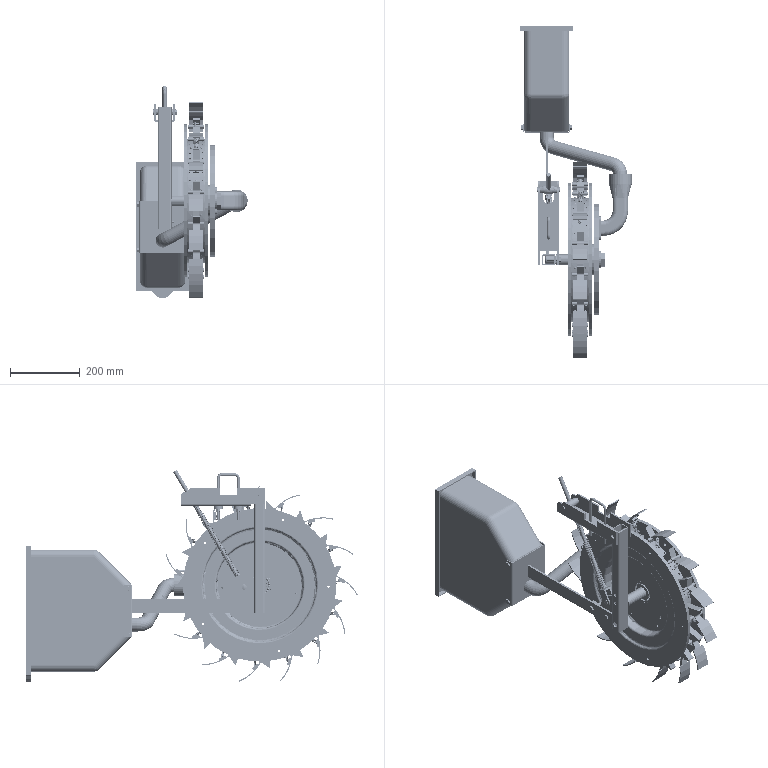Assembly | SolidWorks | mm | 152 component files | 153 solids | 5112 faces | box 318.78 x 951.87 x 608.54 mm | volume 5125266 mm3 | plane 2818 | cylinder 1742 | sphere 196 | torus 194 | cone 118 | spline 44 | commonest cylinder face diameters 3 x287 6 x230 10 x204 0.2 x184 5 x122 5.6 x92 234 x60 9 x58
Bill of materials:
10x25DowelPin | 1 |  | Solid cylindrical pin with a larger-diameter disc head at each end; the outer faces of both heads are slightly domed.
8x50U-Bolt | 1 |  | Round wire or rod bent into a U shape: two straight parallel legs joined by a straight crossbar with rounded bends; one leg is visibly shorter.
hex slotted nuts style 1-grades c gb | 2 |  | Hexagonal nut-like body with a central through bore and radial round-ended slots cut into one end face (castellated form).
hexagon head bolts-full thread gb | 7 |  | Hex-head bolt-like part with a plain cylindrical shank and a chamfered tip.
PullRod | 1 |  | Long slender round rod ending in a forked clevis-style block with two parallel tines, each with a cross hole.
SeedBox | 1 |  | Hollow box-shaped housing or cover with rounded edges, one chamfered (angled) top corner, an open flanged end, and a small cylindrical boss/spigot on one side.
SeedBoxBracket | 1 |  | Sheet-metal bracket: a channel-shaped mounting plate with bent side flanges, plus a long flat arm projecting perpendicular from its face.
SeedBoxCover | 1 |  | Thin flat rectangular plate with a semicircular tab or lobe protruding from the middle of one short edge.
SeederBracket | 1 |  | Rectangular hollow tube post with holes along its length and a flat gusset-like plate with a lobed outline attached near the bottom.
SeederFixingFrame | 1 |  | U-shaped sheet-metal channel bracket with two parallel side plates of stepped height and a connecting web.
16008 Bearing | 2 |  | Ring-shaped assembly resembling a radial ball bearing: concentric inner and outer rings with a ring of spherical elements between them.
cross recessed pan head screws gb | 46 |  | Pan-head screw-like part with a cross-shaped recess in a domed cylindrical head and a plain cylindrical shank.
Duckbill | 15 |  | Thin rectangular base plate curved in one direction, carrying an inclined hollow rectangular column with an open top, a cylindrical knuckle with a bore on the column, and a small tab with an upright cylindrical pin.
DuckbillSpring | 15 |  | Helical coil of round-section wire with a constant coil diameter, roughly 12-13 evenly pitched turns and plain cut ends.
PressingPlate | 15 |  | Thin formed sheet piece: a long curved strip joined at a V-shaped bend to a short straight flange. Hollow cylindrical knuckle(s) sit at the bend, and a rectangular raised pad is on the strip near the bend.
SeedingAxis | 1 |  | Stepped cylindrical pin with a hexagonal head, a thin round collar under the head, a long main shank and a shorter reduced-diameter end section.
SeedingFixingPlate | 1 |  | Large thin circular disc with a central through-bore and stepped concentric cylindrical hub bosses on one face. There is a shallow circular ridge or groove near the rim and two rings of small holes.
SeedingFixingPlateA | 1 |  | Flat annular ring with a stepped cross-section: a thin full-diameter flange plus a thicker layer of smaller outer diameter. It has a large central opening and five small holes on a circle.
SeedingPlate | 1 |  | Thin circular disc with a central round hole and a short cylindrical boss at the center on one face. It has an off-center rounded-square cutout ringed by four small holes, and six small holes near the rim.
SeedingSlot | 15 |  | Complex bracket built around a flat, roughly hexagonal plate with two end lugs that carry cylindrical bosses with through-holes. One side has a rectangular hollow frame or box; the other has an angled hollow channel with a partly cylindrical inner surface and a tapered internal transition.
SeedInlet | 1 |  | Flanged duct: a rectangular flange with rounded corners and four holes leads into a rounded-rectangle duct that bends about 90 degrees, then changes to a larger round section at the far end.
SeedSpoonPlate | 15 |  | Central disc hub with a through-bore. Arms run outward in four directions and end in cylindrical shells of different sizes; some are open semi-cylinders or tubes.
SeedTube | 1 |  | Hollow round tube with two bends forming an offset jog between three straight sections, open at both ends.
ShaftStop | 1 |  | Solid barrel-shaped body bulging in the middle, with a smaller cylindrical spigot at each end and a radial cross-hole through the middle of the body.
single coil spring lock washers heavy gb | 4 |  | Flat annular ring with rectangular cross-section, split by a single narrow radial cut whose faces are angled; resembles a split (helical spring) lock washer.
Spring2 | 1 |  | Long, slender helical coil spring of round wire with constant diameter and many evenly spaced coils; resembles an open-coil compression spring.
Mates:
1. concentric | SeederFixingFrame-1 face at (-210, -105, 2.5) dir (1, 0, 0) r 6 | SeederBracket-1 face at (-20, -105, 2.5) dir (1, 0, 0) r 6
2. coincident | SeederBracket-1 plane at (0, -105, -157.5) dir (1, 0, 0) | assembly plane at (0, 0, 0) dir (1, 0, 0)
3. concentric | SeederFixingFrame-1 face at (-210, -105, 2.5) dir (1, 0, 0) r 6 | hexagon head bolts-full thread gb-1 face at (-5, -105, 2.5) dir (1, 0, 0) r 4
4. coincident | SeederFixingFrame-1 face at (30, 120, 25) dir (1, 0, 0) | hexagon head bolts-full thread gb-1 face at (30, -109.574, -3.45) dir (-1, 0, 0)
5. concentric | SeederFixingFrame-1 face at (-30, 95, 2.5) dir (1, 0, 0) r 7.5 | ShaftStop-1 face at (33, 95, 2.5) dir (-1, 0, 0) r 7.5
6. coincident | ShaftStop-1 plane at (0, 95, 2.5) dir (1, 0, 0) | assembly plane at (0, 0, 0) dir (1, 0, 0)
7. concentric | SeederBracket-1 face at (-2.5, -60.308, -258.214) dir (1, 0, 0) r 5 | PullRod-1 face at (-12.5, -60.308, -258.214) dir (1, 0, 0) r 5
8. concentric | ShaftStop-1 face at (0, 103.444, 16.675) dir (0, -0.5118, -0.8591) r 6 | PullRod-1 face at (0, 138.006, 74.694) dir (0, -0.5118, -0.8591) r 6
9. concentric | PullRod-1 face at (0, 138.006, 74.694) dir (0, -0.5118, -0.8591) r 6 | Spring2-1 sketch segment at (0, -41.116, -225.997) dir (0, 0.5118, 0.8591) r 7.5
10. coincident | PullRod-1 face at (12.5, -30.377, -232.395) dir (0, 0.5118, 0.8591) | Spring2-1 face at (0, -41.116, -225.997) dir (0, -0.5118, -0.8591)
11. concentric | PullRod-1 face at (-12.5, -60.308, -258.214) dir (1, 0, 0) r 5 | 10x25DowelPin-1 face at (14.5, -60.308, -258.214) dir (-1, 0, 0) r 7.5
12. coincident | PullRod-1 face at (12.5, 48.445, -75.652) dir (1, 0, 0) | 10x25DowelPin-1 face at (12.5, -60.308, -258.214) dir (-1, 0, 0)
13. coincident | SeederBracket-1 face at (-2.5, 21.34, -327.5) dir (-1, 0, 0) | SeedBoxBracket-1 face at (-2.5, -90, -292.5) dir (1, 0, 0)
14. concentric | SeederBracket-1 face at (-2.5, -60, -312.5) dir (1, 0, 0) r 5 | SeedBoxBracket-1 face at (-402.5, -60, -312.5) dir (1, 0, 0) r 5
15. concentric | SeederBracket-1 face at (-2.5, 0, -312.5) dir (1, 0, 0) r 5 | SeedBoxBracket-1 face at (-402.5, 0, -312.5) dir (1, 0, 0) r 5
16. concentric | SeedBoxBracket-1 face at (-402.5, -60, -312.5) dir (1, 0, 0) r 5 | hexagon head bolts-full thread gb-2 face at (26.5, -60, -312.5) dir (-1, 0, 0) r 4
17. coincident | SeedBoxBracket-1 face at (-8.5, -90, -292.5) dir (-1, 0, 0) | hexagon head bolts-full thread gb-2 face at (-8.5, -63.753, -319) dir (1, 0, 0)
18. concentric | SeedBoxBracket-1 face at (-402.5, 0, -312.5) dir (1, 0, 0) r 5 | hexagon head bolts-full thread gb-3 face at (26.5, 0, -312.5) dir (-1, 0, 0) r 4
19. coincident | SeedBoxBracket-1 face at (-8.5, -90, -292.5) dir (-1, 0, 0) | hexagon head bolts-full thread gb-3 face at (-8.5, -3.753, -319) dir (1, 0, 0)
20. coincident | SeedBoxBracket-1 face at (57.5, 262.5, -402.5) dir (0, 1, 0) | SeedBox-1 face at (59.5, 262.5, -401.036) dir (0, -1, 0)
21. coincident | SeedBoxBracket-1 face at (59.5, 285, -402.5) dir (-1, 0, 0) | SeedBox-1 face at (59.5, 262.5, -326.036) dir (1, 0, 0)
22. coincident | SeedBoxBracket-1 face at (-68.5, 264.5, -402.5) dir (0, 0, -1) | SeedBox-1 edge at (39.5, 263.964, -402.5) dir (-1, 0, 0)
23. coincident | SeedBoxBracket-1 face at (62, 285, -402.5) dir (1, 0, 0) | hexagon head bolts-full thread gb-4 face at (62, 279.324, -256.55) dir (-1, 0, 0)
24. concentric | SeedBoxBracket-1 face at (-73, 274.75, -262.5) dir (1, 0, 0) r 4.5 | hexagon head bolts-full thread gb-4 face at (27, 274.75, -262.5) dir (1, 0, 0) r 4
25. concentric | SeedBoxBracket-1 face at (-73, 274.75, -392.5) dir (1, 0, 0) r 4.5 | hexagon head bolts-full thread gb-5 face at (27, 274.75, -392.5) dir (1, 0, 0) r 4
26. coincident | SeedBoxBracket-1 face at (62, 285, -402.5) dir (1, 0, 0) | hexagon head bolts-full thread gb-5 face at (62, 270.176, -398.45) dir (-1, 0, 0)
27. concentric | SeedBoxBracket-1 face at (-73, 274.75, -392.5) dir (1, 0, 0) r 4.5 | hexagon head bolts-full thread gb-6 face at (-38, 274.75, -392.5) dir (-1, 0, 0) r 4
28. coincident | SeedBoxBracket-1 face at (-73, 264.5, -402.5) dir (-1, 0, 0) | hexagon head bolts-full thread gb-6 face at (-73, 270.997, -399) dir (1, 0, 0)
29. concentric | SeedBoxBracket-1 face at (-73, 274.75, -262.5) dir (1, 0, 0) r 4.5 | hexagon head bolts-full thread gb-7 face at (-38, 274.75, -262.5) dir (-1, 0, 0) r 4
30. coincident | SeedBoxBracket-1 face at (-73, 264.5, -402.5) dir (-1, 0, 0) | hexagon head bolts-full thread gb-7 face at (-73, 270.997, -269) dir (1, 0, 0)
31. coincident | SeedBox-1 face at (59.5, 562.5, -151.036) dir (0, 1, 0) | SeedBoxCover-1 face at (-5.5, 562.5, -326.036) dir (0, -1, 0)
32. distance | SeedBox-1 face at (64.5, 556.5, -171.036) dir (1, 0, 0) | SeedBoxCover-1 face at (67, 565, -141.036) dir (-1, 0, 0)
33. distance | SeedBoxCover-1 face at (69.5, 565, -143.536) dir (0, 0, -1) | SeedBox-1 face at (-50.5, 556.5, -146.036) dir (0, 0, 1)
34. concentric | SeederFixingFrame-1 face at (0, 14, -260) dir (0, 0, 1) r 5 | 8x50U-Bolt-1 face at (0, 14, 54) dir (0, 0, -1) r 4
35. concentric | SeederFixingFrame-1 face at (0, -44, -260) dir (0, 0, 1) r 5 | 8x50U-Bolt-1 face at (0, -44, 54) dir (0, 0, -1) r 4
36. distance | 8x50U-Bolt-1 face at (0, -34, 64) dir (0, 1, 0) r 4 | SeederFixingFrame-1 face at (-210, -40, 5) dir (0, 0, 1)
37. parallel | SeederFixingFrame-1 face at (25, -120, -20) dir (0, -1, 0) | SeederBracket-1 face at (-15, -120, 17.5) dir (0, -1, 0)
38. concentric | SeedBoxBracket-1 edge at (-5.5, 260, -366.036) dir (0, 1, 0) r 20 | SeedTube-1 edge at (-5.5, 262.5, -366.036) dir (0, -1, 0) r 18
39. coincident | SeedBox-1 face at (59.5, 262.5, -401.036) dir (0, -1, 0) | SeedTube-1 face at (-5.5, 262.5, -366.036) dir (0, 1, 0)
40. concentric | SeedTube-1 face at (205.776, 72.5, -252.184) dir (0, 1, 0) r 20 | SeedingAssemblyA-1/SeedInlet-1 face at (205.776, 141, -252.184) dir (0, -1, 0) r 30.5
41. parallel | SeederBracket-1 face at (20, -115, 17.5) dir (1, 0, 0) | SeedingAssemblyA-1/SeedingFixingPlate-1 face at (55.776, 19.599, -70.868) dir (-1, 0, 0)
42. concentric | 8x50U-Bolt-1 face at (0, 14, 54) dir (0, 0, -1) r 4 | hex slotted nuts style 1-grades c gb-1 face at (0, 14, -34.6) dir (0, 0, -1) r 4
43. concentric | 8x50U-Bolt-1 face at (0, -44, 54) dir (0, 0, -1) r 4 | hex slotted nuts style 1-grades c gb-2 face at (0, -44, -34.6) dir (0, 0, -1) r 4
44. concentric | 8x50U-Bolt-1 face at (0, 14, 54) dir (0, 0, -1) r 4 | single coil spring lock washers heavy gb-1 face at (0, 14, -29.8) dir (0, 0, -1) r 8
45. concentric | single coil spring lock washers heavy gb-1 face at (0, 14, -29.8) dir (0, 0, -1) r 13.3 | single coil spring lock washers heavy gb-2 face at (0, 14, -29.8) dir (0, 0, 1) r 8
46. coincident | single coil spring lock washers heavy gb-1 face at (0, 14, -29.8) dir (0, 0, 1) | single coil spring lock washers heavy gb-2 face at (0, 14, -29.8) dir (0, 0, -1)
47. concentric | 8x50U-Bolt-1 face at (0, -44, 54) dir (0, 0, -1) r 4 | single coil spring lock washers heavy gb-3 face at (0, -44, -25) dir (0, 0, -1) r 8
48. concentric | 8x50U-Bolt-1 face at (0, -44, 54) dir (0, 0, -1) r 4 | single coil spring lock washers heavy gb-4 face at (0, -44, -29.8) dir (0, 0, -1) r 8
49. coincident | SeederFixingFrame-1 face at (-25, 120, -25) dir (0, 0, -1) | single coil spring lock washers heavy gb-2 face at (0, 14, -25) dir (0, 0, 1)
50. coincident | hex slotted nuts style 1-grades c gb-1 face at (-3.753, 7.5, -34.6) dir (0, 0, 1) | single coil spring lock washers heavy gb-1 face at (0, 14, -34.6) dir (0, 0, -1)
51. concentric | single coil spring lock washers heavy gb-3 face at (0, -44, -25) dir (0, 0, -1) r 13.3 | single coil spring lock washers heavy gb-4 face at (0, -44, -29.8) dir (0, 0, -1) r 13.3
52. concentric | 8x50U-Bolt-1 face at (0, -44, 54) dir (0, 0, -1) r 4 | single coil spring lock washers heavy gb-3 face at (0, -44, -25) dir (0, 0, -1) r 13.3
53. coincident | SeederFixingFrame-1 face at (-25, 120, -25) dir (0, 0, -1) | single coil spring lock washers heavy gb-3 face at (0, -44, -25) dir (0, 0, 1)
54. coincident | single coil spring lock washers heavy gb-3 edge at (0, -44, -29.8) dir (0, 0, -1) r 13.3 | single coil spring lock washers heavy gb-4 face at (0, -44, -29.8) dir (0, 0, 1)
55. coincident | hex slotted nuts style 1-grades c gb-2 face at (-4.455, -50.041, -34.6) dir (0, 0, 1) | single coil spring lock washers heavy gb-4 face at (0, -44, -34.6) dir (0, 0, -1)
56. coincident | Duckbill-1 face at (250.64, -48.759, 312.92) dir (0.9914, -0.1306, 0) | DuckbillSpring-1 plane at (248.028, -68.588, 347.545) dir (0.9914, -0.1306, 0)
57. coincident | Duckbill-1 axis at (257.942, -69.894, 347.545) dir (-0.9914, 0.1306, 0) | DuckbillSpring-1 axis at (244.715, -68.151, 347.545) dir (0.9914, -0.1306, 0)
58. concentric | Duckbill-1 face at (269.261, -54.238, 338.045) dir (0, 0, 1) r 4.5 | PressingPlate-1 face at (269.261, -54.238, 370.045) dir (0, 0, -1) r 2.5
59. coincident | Duckbill-1 face at (292.362, -54.254, 338.045) dir (0, 0, -1) | PressingPlate-1 face at (269.261, -54.238, 338.045) dir (0, 0, 1)
60. coincident | SeedingFixingPlate-1 face at (55.985, -11.017, 338.5) dir (0, 0, 1) | 16008Bearing-1 face at (89.402, -4.75, 338.5) dir (0, 0, -1)
61. concentric | SeedingFixingPlate-1 face at (55.985, -11.017, 338.5) dir (0, 0, 1) r 34 | 16008Bearing-1 face at (55.985, -11.017, 351.711) dir (0, 0, 1) r 34
62. coincident | SeedingFixingPlate-1 face at (55.985, -11.017, 316.5) dir (0, 0, -1) | 16008Bearing-2 face at (89.402, -4.75, 316.5) dir (0, 0, 1)
63. concentric | SeedingFixingPlate-1 face at (242.152, -76.955, 372.5) dir (0, 0, -1) r 3.4 | SeedingFixingPlateA-1 face at (242.152, -76.955, 337.5) dir (0, 0, -1) r 4.5
64. coincident | Duckbill-11 face at (55.985, -11.017, -308.055) dir (-0.8242, -0.5664, 0) | SeedingFixingPlateA-1 plane at (55.985, -11.017, 322.5) dir (0.8242, 0.5664, 0)
65. coincident | SeedingPlate-1 face at (55.985, -11.017, 292.5) dir (0, 0, -1) | SeedInlet-1 face at (40.985, 68.983, 292.5) dir (0, 0, 1)
66. concentric | SeedingPlate-1 face at (85.985, 103.983, 292.5) dir (0, 0, -1) r 2.5 | SeedInlet-1 face at (85.985, 103.983, 292.5) dir (0, 0, -1) r 3.25
67. concentric | SeedingPlate-1 face at (85.985, 53.983, 292.5) dir (0, 0, -1) r 2.5 | SeedInlet-1 face at (85.985, 53.983, 292.5) dir (0, 0, -1) r 3.25
68. coincident | Duckbill-5 face at (24.262, -185.945, 340.045) dir (-0.9724, 0.2335, 0) | SeedingSlot-1 face at (23.561, -188.862, 355.045) dir (0.9724, -0.2335, 0)
69. coincident | Duckbill-4 face at (98.154, -183.725, 355.045) dir (0, 0, -1) | SeedingSlot-1 face at (23.561, -188.862, 355.045) dir (0, 0, 1)
70. concentric | Duckbill-5 face at (24.253, -250.22, 347.545) dir (0.2335, 0.9724, 0) r 1.5 | SeedSpoonPlate-1 face at (40.832, -181.183, 347.545) dir (-0.2335, -0.9724, 0) r 1.5
71. distance | SeedSpoonPlate-1 face at (40.365, -183.128, 347.545) dir (-0.2335, -0.9724, 0) | Duckbill-5 face at (55.985, -11.017, 322.595) dir (0, 0, 1) r 175
72. parallel | SeedingSlot-1 face at (24.498, -182.301, 351.303) dir (0, 0, -1) | SeedSpoonPlate-1 face at (34.997, -179.782, 346.545) dir (0, 0, -1)
73. concentric | Duckbill-5 face at (-0.05591, -244.383, 332.545) dir (0.2335, 0.9724, 0) r 1.5 | SeedingSlot-1 face at (14.248, -184.819, 332.545) dir (0.2335, 0.9724, 0) r 1.5
74. concentric | Duckbill-5 face at (-0.05591, -244.383, 362.545) dir (0.2335, 0.9724, 0) r 1.5 | SeedingSlot-1 face at (14.248, -184.819, 362.545) dir (0.2335, 0.9724, 0) r 1.5
75. concentric | Duckbill-5 face at (24.253, -250.22, 347.545) dir (0.2335, 0.9724, 0) r 1.5 | cross recessed pan head screws gb-7 face at (39.341, -187.391, 347.545) dir (0.2335, 0.9724, 0) r 1.5
76. tangent | Duckbill-6 face at (55.985, -11.017, 322.595) dir (0, 0, 1) r 177.5 | cross recessed pan head screws gb-7 face at (37.165, -189.044, 348.043) dir (0.2335, 0.9724, 0)
77. concentric | Duckbill-5 face at (-0.05591, -244.383, 332.545) dir (0.2335, 0.9724, 0) r 1.5 | cross recessed pan head screws gb-6 face at (15.032, -181.553, 332.545) dir (0.2335, 0.9724, 0) r 1.5
78. concentric | Duckbill-5 face at (-0.05591, -244.383, 362.545) dir (0.2335, 0.9724, 0) r 1.5 | cross recessed pan head screws gb-5 face at (15.032, -181.553, 362.545) dir (0.2335, 0.9724, 0) r 1.5
79. tangent | Duckbill-5 face at (55.985, -11.017, 322.595) dir (0, 0, 1) r 177.5 | cross recessed pan head screws gb-5 face at (16.196, -184.009, 363.12) dir (0.2335, 0.9724, 0)
80. tangent | Duckbill-5 face at (55.985, -11.017, 322.595) dir (0, 0, 1) r 177.5 | cross recessed pan head screws gb-6 face at (12.879, -183.212, 333.119) dir (0.2335, 0.9724, 0)
81. distance | SeedingSlot-1 face at (15.238, -180.693, 332.545) dir (-0.2335, -0.9724, 0) | cross recessed pan head screws gb-6 face at (12.879, -183.212, 333.119) dir (0.2335, 0.9724, 0)
82. concentric | SeedingPlate-1 face at (55.985, -11.017, 292.5) dir (0, 0, 1) r 15 | SeedingAxis-1 face at (55.985, -11.017, 417.5) dir (0, 0, -1) r 15
83. coincident | SeedingPlate-1 face at (55.985, -11.017, 292.5) dir (0, 0, -1) | SeedingAxis-1 face at (55.985, -11.017, 292.5) dir (0, 0, 1)